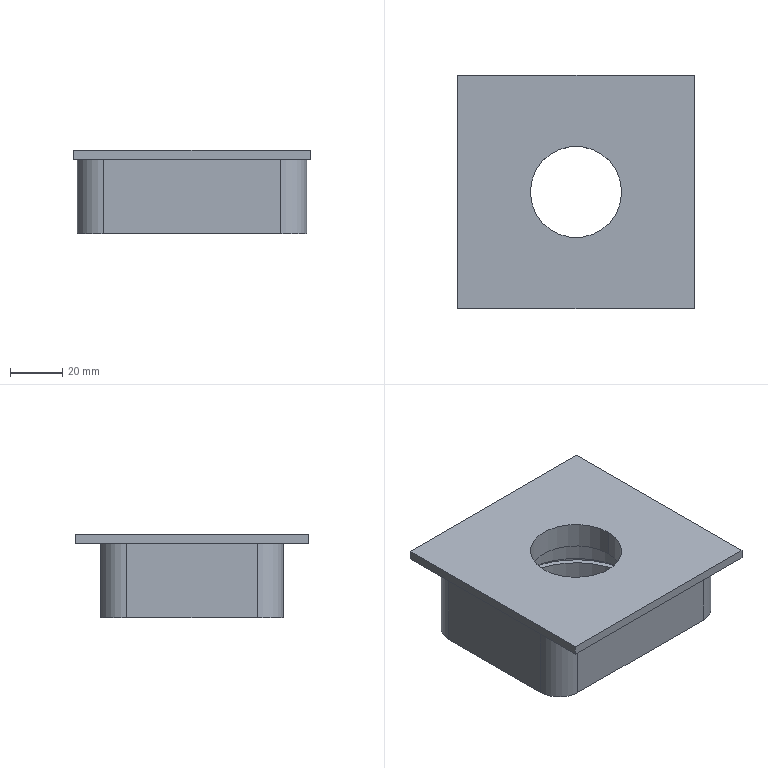Component | SolidWorks | 12AEncoderWheel-1_12AEncoderAxisFrontBaffle-1 | 1 solid | 42 faces | box 90.5 x 89.5 x 32 mm | volume 133103 mm3 | cylinder 20 | plane 14 | cone 8 | commonest cylinder face diameters 8.5 x8 55 x4 20 x4 59 x2 35 x2
build123d program:
from build123d import *

# Parameters (mm, degrees)
SKETCH1_W              = 89.5
SKETCH1_H              = 90.5
BOSS_EXTRUDE1_DEPTH    = 3.5
BOSS_EXTRUDE2_DEPTH    = 28.5
SKETCH3_R              = 27.5
CUT_EXTRUDE1_DEPTH     = 22
SKETCH4_R              = 17.5
CUT_EXTRUDE2_DEPTH     = 72.233
M10_TAPPED_HOLE1_D     = 8.5
M10_TAPPED_HOLE1_DEPTH = 24.5
M10_TAPPED_HOLE1_TIP   = 2.554
CUT_EXTRUDE3_START     = 2
SKETCH7_R              = 29.5
SKETCH7_R_2            = 27.5
CUT_EXTRUDE3_DEPTH     = 2


with BuildPart() as part:
    # Sketch1 → Boss-Extrude1 (new body)
    with BuildSketch(Plane(origin=(0, 0, 0), x_dir=(1, 0, 0), z_dir=(0, 1, 0))):
        Rectangle(SKETCH1_W, SKETCH1_H)
    extrude(amount=BOSS_EXTRUDE1_DEPTH)

    # Sketch2 → Boss-Extrude2 (add)
    with BuildSketch(Plane(origin=(0, 3.5, 0), x_dir=(1, 0, 0), z_dir=(0, 1, 0))):
        with BuildLine():
            Line((-25, 44), (25, 44))
            ThreePointArc((25, 44), (32.071, 41.071), (35, 34))
            Line((35, 34), (35, -34))
            ThreePointArc((35, -34), (32.071, -41.071), (25, -44))
            Line((25, -44), (-25, -44))
            ThreePointArc((-25, -44), (-32.071, -41.071), (-35, -34))
            Line((-35, -34), (-35, 34))
            ThreePointArc((-35, 34), (-32.071, 41.071), (-25, 44))
        make_face()
    extrude(amount=BOSS_EXTRUDE2_DEPTH)

    # Sketch3 → Cut-Extrude1 (cut)
    with BuildSketch(Plane(origin=(0, 32, 0), x_dir=(1, 0, 0), z_dir=(0, 1, 0))):
        with Locations(Location((0, 0, 0), (0, 0, 270))):
            Circle(SKETCH3_R)
    extrude(amount=-CUT_EXTRUDE1_DEPTH, mode=Mode.SUBTRACT)

    # Sketch4 → Cut-Extrude2 (cut, through all)
    with BuildSketch(Plane.XZ):
        with Locations(Location((0, 0, 0), (0, 0, 270))):
            Circle(SKETCH4_R)
    extrude(amount=-CUT_EXTRUDE2_DEPTH, mode=Mode.SUBTRACT)

    # M10 Tapped Hole1
    with Locations(Plane(origin=(0, 32, 0), x_dir=(1, 0, 0), z_dir=(0, 1, 0))):
        with Locations((-27, 36), (27, 36), (27, -36), (-27, -36)):
            Hole(M10_TAPPED_HOLE1_D / 2, depth=M10_TAPPED_HOLE1_DEPTH)
            with Locations((0, 0, -(M10_TAPPED_HOLE1_DEPTH + M10_TAPPED_HOLE1_TIP / 2))):  # 118° drill point
                Cone(0, M10_TAPPED_HOLE1_D / 2, M10_TAPPED_HOLE1_TIP, mode=Mode.SUBTRACT)

    # Sketch7 → Cut-Extrude3 (cut)
    with BuildSketch(Plane(origin=(0, 23, 0), x_dir=(1, 0, 0), z_dir=(0, 1, 0)).offset(CUT_EXTRUDE3_START)):
        with Locations(Location((0, 0, 0), (0, 0, 270))):
            Circle(SKETCH7_R)
        with Locations(Location((0, 0, 0), (0, 0, 270))):
            Circle(SKETCH7_R_2, mode=Mode.SUBTRACT)
    extrude(amount=-CUT_EXTRUDE3_DEPTH, mode=Mode.SUBTRACT)


solid = part.part

# Placed as in the assembly
solid = solid.moved(Location((120.894, 147.181, 17.75), (-90, 90, 0)))